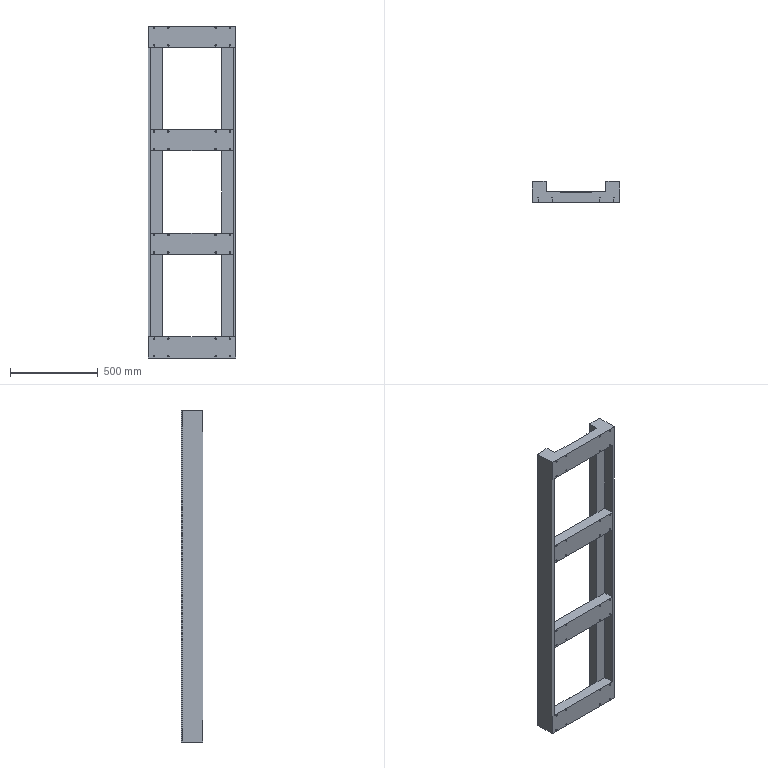Component | SolidWorks | MainBeam-1 | 1 solid | 330 faces | volume 34231263 mm3 | cylinder 140 | cone 138 | plane 52 | commonest cylinder face diameters 10.2 x72 8.5 x64 14.5 x2 20 x2